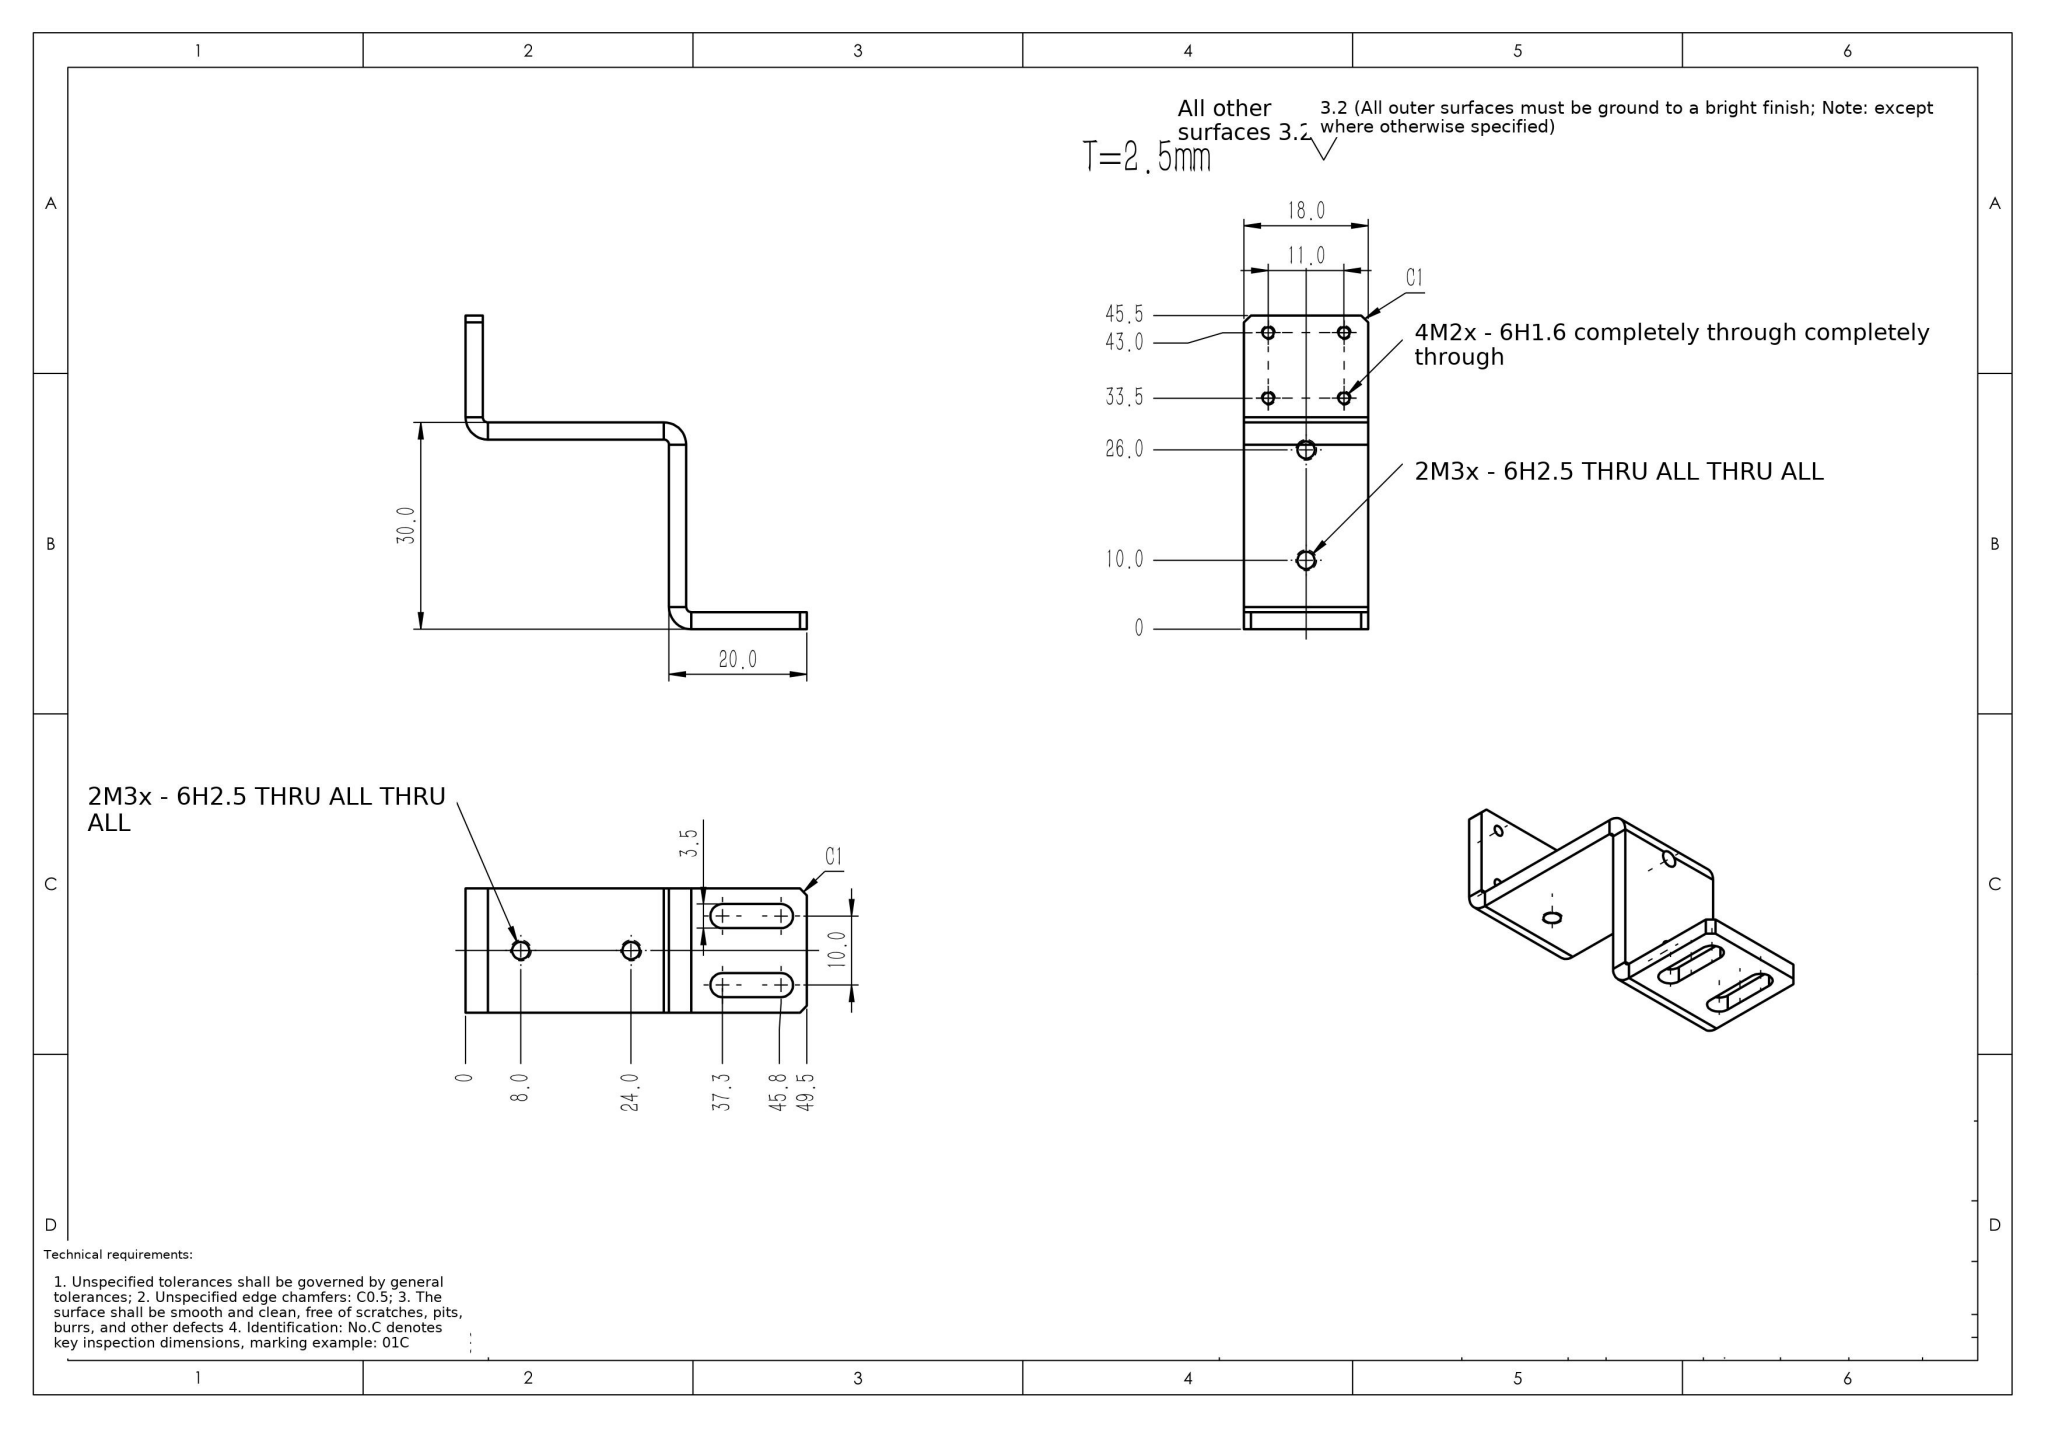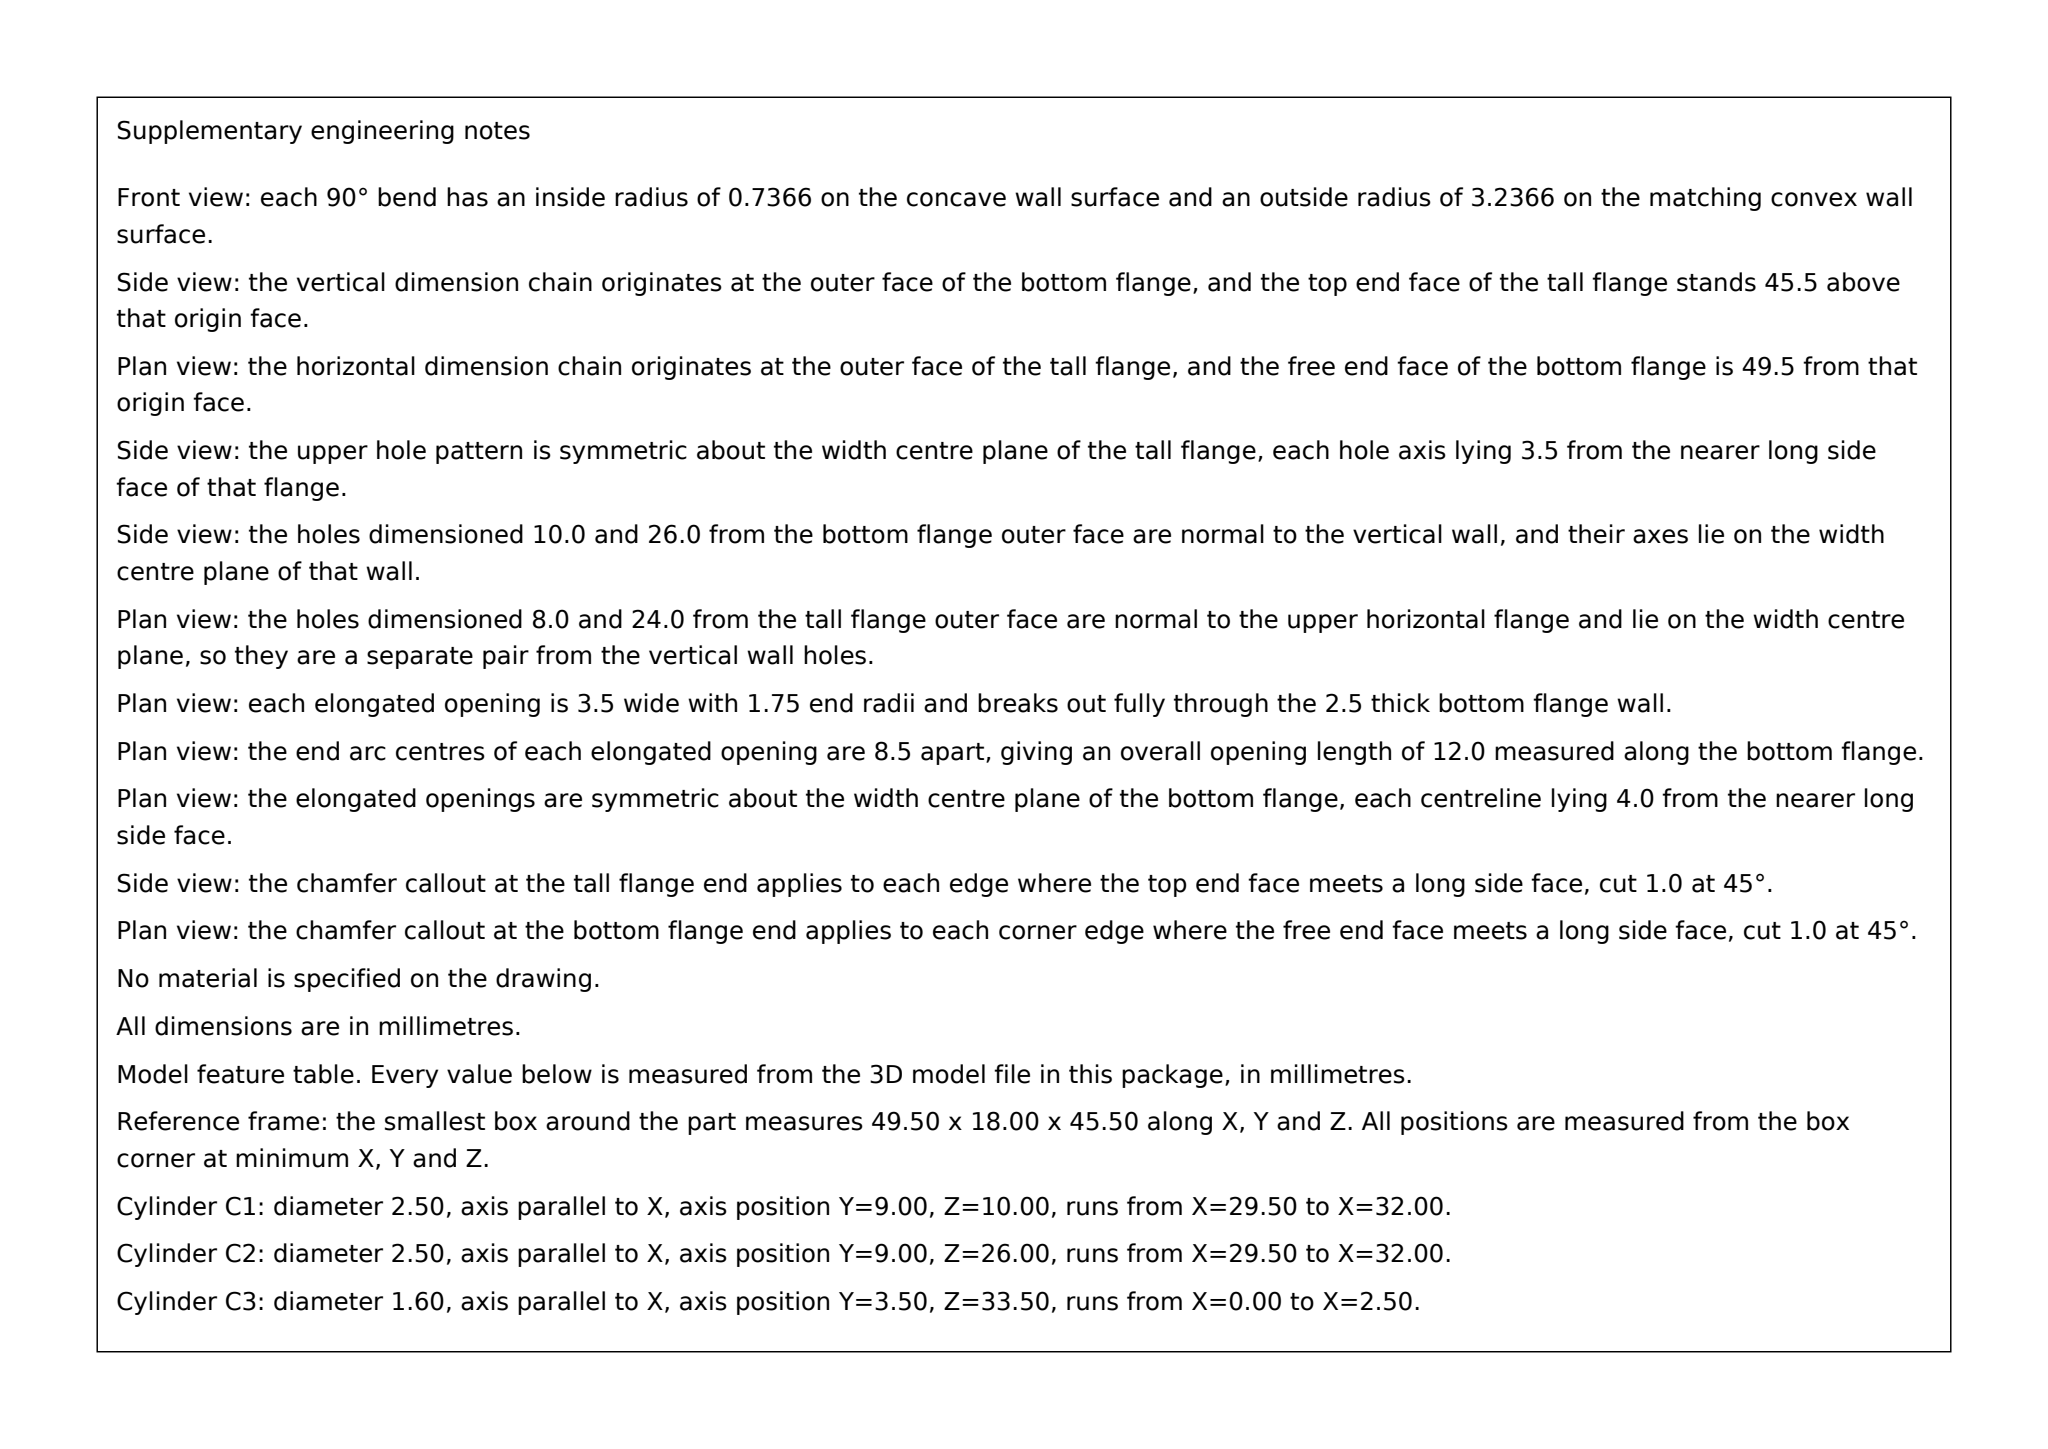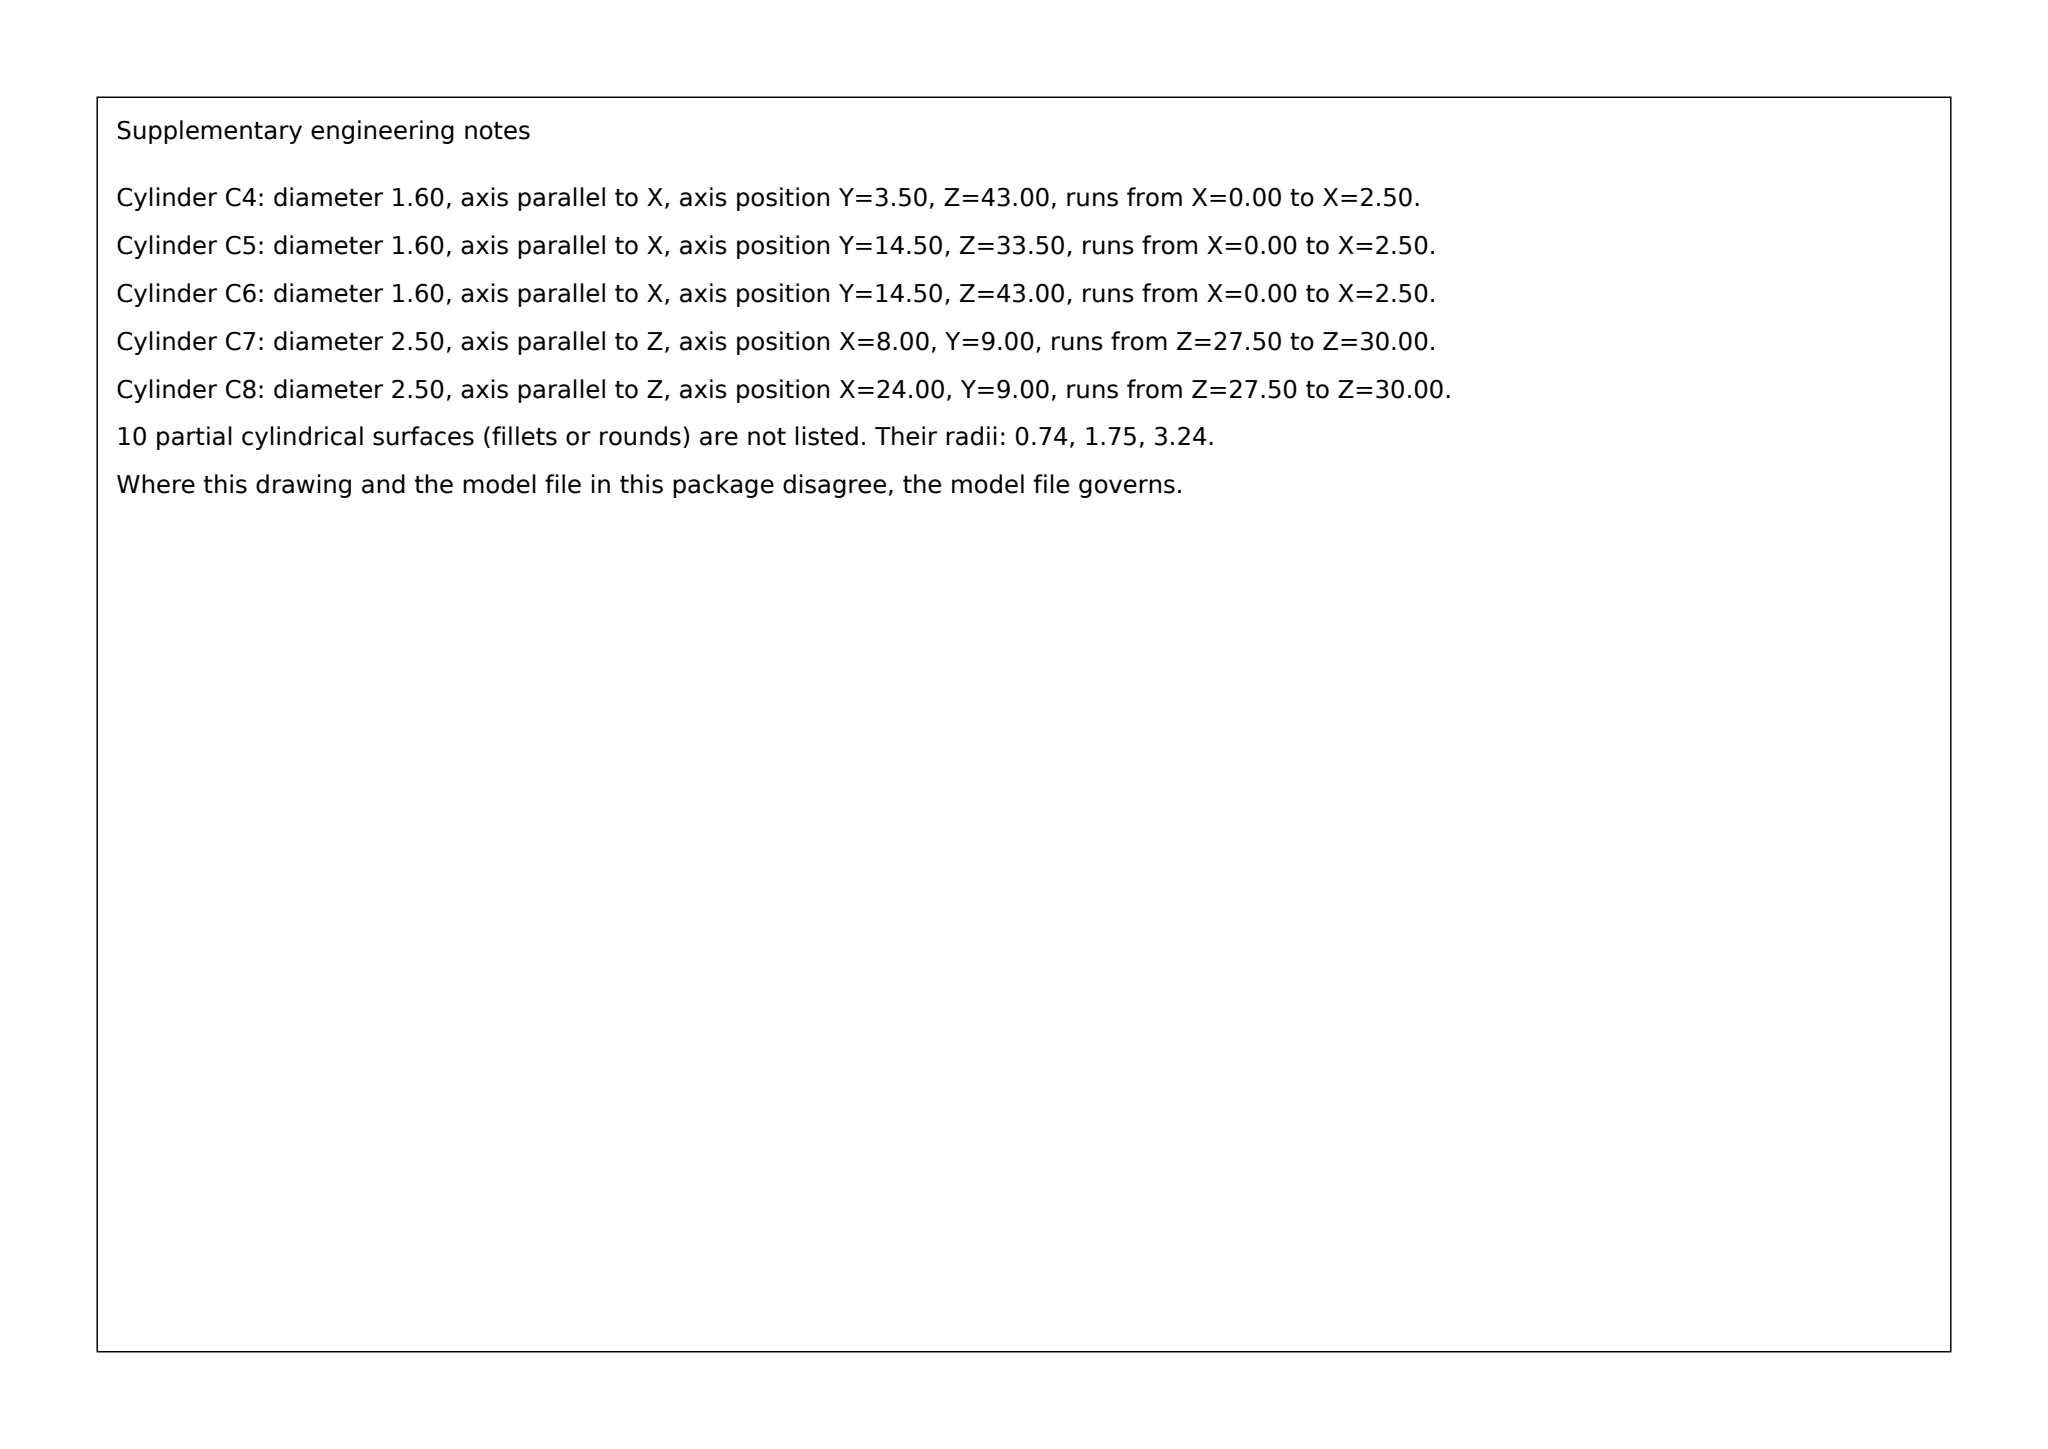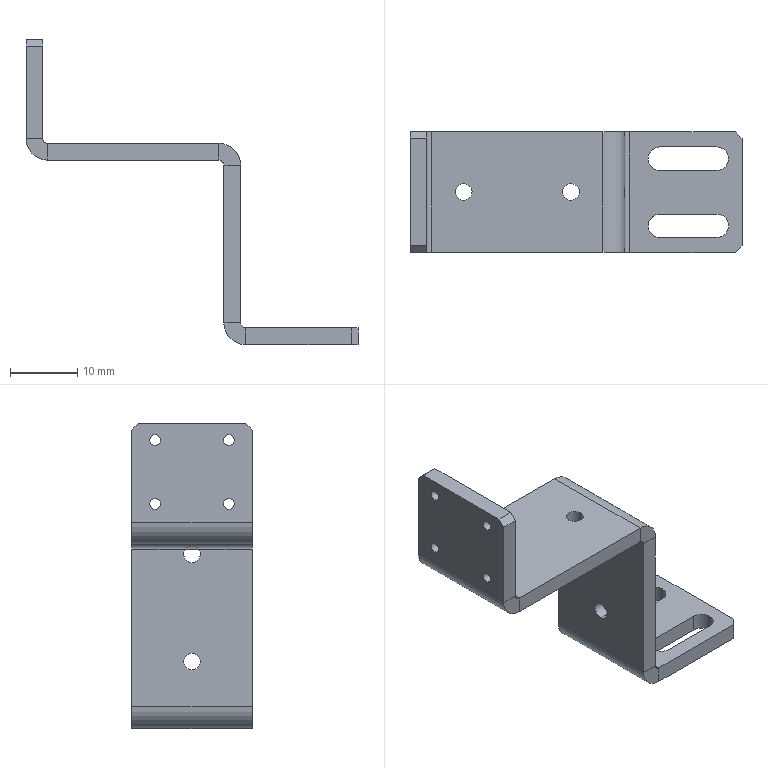Part | SolidWorks | mm | 1 solid | 61 faces | box 49.5 x 18 x 45.5 mm | volume 3776 mm3 | plane 33 | cylinder 28 | commonest cylinder face diameters 2.5 x8 1.6 x8 3.5 x6 6.473 x3 1.473 x3
Drawing notes:
ALL 3 BENDS: INSIDE R0.74, OUTSIDE R3.24, T=2.5 | from the solid: cylinders dia 1.473 (R0.7365) and dia 6.473 (R3.236), axis y, length 18.0, 3 each at bend corners (3.24,30.74), (28.76,26.76), (32.74,3.24)